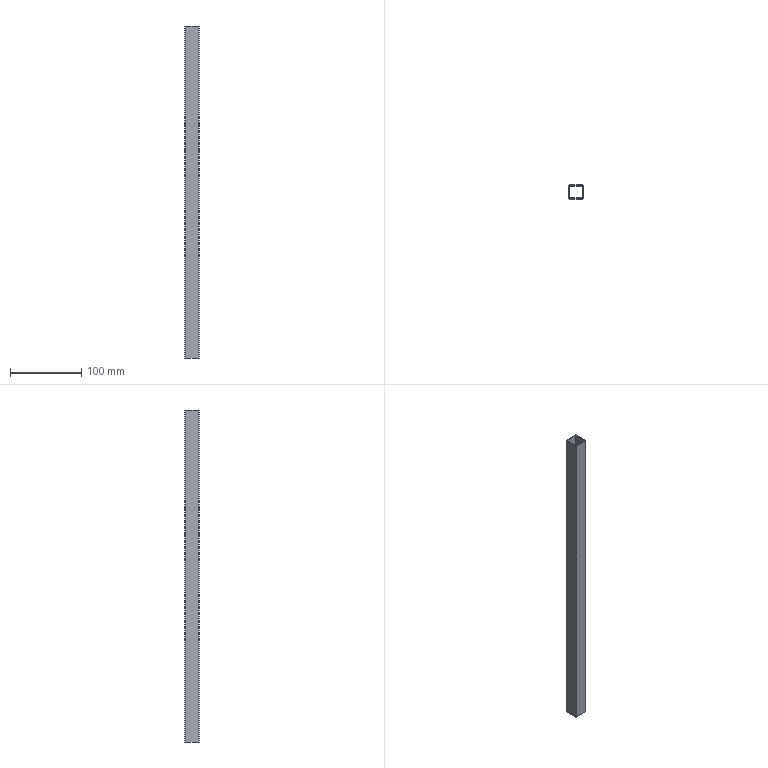Component | SolidWorks | Stiffener-1 | 1 solid | 14 faces | box 20 x 20 x 467.6 mm | volume 41795 mm3 | plane 10 | cylinder 4 | commonest cylinder face diameters 2 x4
build123d program:
from build123d import *

# Parameters (mm, degrees)
SKETCH1_W           = 17.6
SKETCH1_H           = 17.6
BOSS_EXTRUDE1_DEPTH = 467.6


with BuildPart() as part:
    # Sketch1 → Boss-Extrude1 (new body)
    with BuildSketch(Plane.XY):
        with BuildLine():
            Line((-75.47, 58.704), (-57.47, 58.704))
            ThreePointArc((-57.47, 58.704), (-56.763, 58.411), (-56.47, 57.704))
            Line((-56.47, 57.704), (-56.47, 39.704))
            ThreePointArc((-56.47, 39.704), (-56.763, 38.997), (-57.47, 38.704))
            Line((-57.47, 38.704), (-75.47, 38.704))
            ThreePointArc((-75.47, 38.704), (-76.177, 38.997), (-76.47, 39.704))
            Line((-76.47, 39.704), (-76.47, 57.704))
            ThreePointArc((-76.47, 57.704), (-76.177, 58.411), (-75.47, 58.704))
        make_face()
        with Locations((-66.47, 48.704)):
            Rectangle(SKETCH1_W, SKETCH1_H, mode=Mode.SUBTRACT)
    extrude(amount=BOSS_EXTRUDE1_DEPTH)


solid = part.part

# Placed as in the assembly
solid = solid.moved(Location((274.97, 197.296, -115.8), (0, 0, 0)))
STEP:
#1=CARTESIAN_POINT('',(8.563,9.291,13.85));
#2=VERTEX_POINT('',#1);
#3=CARTESIAN_POINT('',(8.602,9.331,13.85));
#4=VERTEX_POINT('',#3);
#5=CARTESIAN_POINT('',(8.563,9.331,13.85));
#6=DIRECTION('',(-0.,0.,1.));
#7=DIRECTION('',(-1.,0.,0.));
#8=AXIS2_PLACEMENT_3D('',#5,#6,#7);
#9=CIRCLE('',#8,0.03937);
#10=EDGE_CURVE('',#2,#4,#9,.T.);
#11=ORIENTED_EDGE('',*,*,#10,.T.);
#12=CARTESIAN_POINT('',(8.602,10.039,13.85));
#13=VERTEX_POINT('',#12);
#14=CARTESIAN_POINT('',(8.602,9.331,13.85));
#15=DIRECTION('',(-0.,1.,-0.));
#16=VECTOR('',#15,39.37);
#17=LINE('',#14,#16);
#18=EDGE_CURVE('',#4,#13,#17,.T.);
#19=ORIENTED_EDGE('',*,*,#18,.T.);
#20=CARTESIAN_POINT('',(8.563,10.079,13.85));
#21=VERTEX_POINT('',#20);
#22=CARTESIAN_POINT('',(8.563,10.039,13.85));
#23=DIRECTION('',(-0.,0.,1.));
#24=DIRECTION('',(1.,0.,0.));
#25=AXIS2_PLACEMENT_3D('',#22,#23,#24);
#26=CIRCLE('',#25,0.03937);
#27=EDGE_CURVE('',#13,#21,#26,.T.);
#28=ORIENTED_EDGE('',*,*,#27,.T.);
#29=CARTESIAN_POINT('',(7.854,10.079,13.85));
#30=VERTEX_POINT('',#29);
#31=CARTESIAN_POINT('',(8.563,10.079,13.85));
#32=DIRECTION('',(-1.,0.,-0.));
#33=VECTOR('',#32,39.37);
#34=LINE('',#31,#33);
#35=EDGE_CURVE('',#21,#30,#34,.T.);
#36=ORIENTED_EDGE('',*,*,#35,.T.);
#37=CARTESIAN_POINT('',(7.815,10.039,13.85));
#38=VERTEX_POINT('',#37);
#39=CARTESIAN_POINT('',(7.854,10.039,13.85));
#40=DIRECTION('',(-0.,0.,1.));
#41=DIRECTION('',(-1.,0.,0.));
#42=AXIS2_PLACEMENT_3D('',#39,#40,#41);
#43=CIRCLE('',#42,0.03937);
#44=EDGE_CURVE('',#30,#38,#43,.T.);
#45=ORIENTED_EDGE('',*,*,#44,.T.);
#46=CARTESIAN_POINT('',(7.815,9.331,13.85));
#47=VERTEX_POINT('',#46);
#48=CARTESIAN_POINT('',(7.815,9.331,13.85));
#49=DIRECTION('',(-0.,-1.,0.));
#50=VECTOR('',#49,39.37);
#51=LINE('',#48,#50);
#52=EDGE_CURVE('',#38,#47,#51,.T.);
#53=ORIENTED_EDGE('',*,*,#52,.T.);
#54=CARTESIAN_POINT('',(7.854,9.291,13.85));
#55=VERTEX_POINT('',#54);
#56=CARTESIAN_POINT('',(7.854,9.331,13.85));
#57=DIRECTION('',(-0.,0.,1.));
#58=DIRECTION('',(-1.,0.,0.));
#59=AXIS2_PLACEMENT_3D('',#56,#57,#58);
#60=CIRCLE('',#59,0.03937);
#61=EDGE_CURVE('',#47,#55,#60,.T.);
#62=ORIENTED_EDGE('',*,*,#61,.T.);
#63=CARTESIAN_POINT('',(8.563,9.291,13.85));
#64=DIRECTION('',(1.,-0.,0.));
#65=VECTOR('',#64,39.37);
#66=LINE('',#63,#65);
#67=EDGE_CURVE('',#55,#2,#66,.T.);
#68=ORIENTED_EDGE('',*,*,#67,.T.);
#69=EDGE_LOOP('',(#11,#19,#28,#36,#45,#53,#62,#68));
#70=FACE_OUTER_BOUND('',#69,.T.);
#71=CARTESIAN_POINT('',(8.555,9.339,13.85));
#72=VERTEX_POINT('',#71);
#73=CARTESIAN_POINT('',(8.555,10.031,13.85));
#74=VERTEX_POINT('',#73);
#75=CARTESIAN_POINT('',(8.555,9.339,13.85));
#76=DIRECTION('',(0.,1.,-0.));
#77=VECTOR('',#76,39.37);
#78=LINE('',#75,#77);
#79=EDGE_CURVE('',#72,#74,#78,.T.);
#80=ORIENTED_EDGE('',*,*,#79,.F.);
#81=CARTESIAN_POINT('',(7.862,9.339,13.85));
#82=VERTEX_POINT('',#81);
#83=CARTESIAN_POINT('',(8.555,9.339,13.85));
#84=DIRECTION('',(1.,-0.,0.));
#85=VECTOR('',#84,39.37);
#86=LINE('',#83,#85);
#87=EDGE_CURVE('',#82,#72,#86,.T.);
#88=ORIENTED_EDGE('',*,*,#87,.F.);
#89=CARTESIAN_POINT('',(7.862,10.031,13.85));
#90=VERTEX_POINT('',#89);
#91=CARTESIAN_POINT('',(7.862,9.339,13.85));
#92=DIRECTION('',(-0.,-1.,0.));
#93=VECTOR('',#92,39.37);
#94=LINE('',#91,#93);
#95=EDGE_CURVE('',#90,#82,#94,.T.);
#96=ORIENTED_EDGE('',*,*,#95,.F.);
#97=CARTESIAN_POINT('',(8.555,10.031,13.85));
#98=DIRECTION('',(-1.,0.,-0.));
#99=VECTOR('',#98,39.37);
#100=LINE('',#97,#99);
#101=EDGE_CURVE('',#74,#90,#100,.T.);
#102=ORIENTED_EDGE('',*,*,#101,.F.);
#103=EDGE_LOOP('',(#80,#88,#96,#102));
#104=FACE_BOUND('',#103,.T.);
#105=CARTESIAN_POINT('',(8.563,9.331,13.85));
#106=DIRECTION('',(-0.,0.,1.));
#107=DIRECTION('',(-1.,0.,-0.));
#108=AXIS2_PLACEMENT_3D('',#105,#106,#107);
#109=PLANE('',#108);
#110=ADVANCED_FACE('',(#70,#104),#109,.T.);
#111=CARTESIAN_POINT('',(8.563,9.291,-4.559));
#112=VERTEX_POINT('',#111);
#113=CARTESIAN_POINT('',(8.602,9.331,-4.559));
#114=VERTEX_POINT('',#113);
#115=CARTESIAN_POINT('',(8.563,9.331,-4.559));
#116=DIRECTION('',(-0.,0.,1.));
#117=DIRECTION('',(-1.,0.,0.));
#118=AXIS2_PLACEMENT_3D('',#115,#116,#117);
#119=CIRCLE('',#118,0.03937);
#120=EDGE_CURVE('',#112,#114,#119,.T.);
#121=ORIENTED_EDGE('',*,*,#120,.F.);
#122=CARTESIAN_POINT('',(7.854,9.291,-4.559));
#123=VERTEX_POINT('',#122);
#124=CARTESIAN_POINT('',(8.563,9.291,-4.559));
#125=DIRECTION('',(1.,-0.,0.));
#126=VECTOR('',#125,39.37);
#127=LINE('',#124,#126);
#128=EDGE_CURVE('',#123,#112,#127,.T.);
#129=ORIENTED_EDGE('',*,*,#128,.F.);
#130=CARTESIAN_POINT('',(7.815,9.331,-4.559));
#131=VERTEX_POINT('',#130);
#132=CARTESIAN_POINT('',(7.854,9.331,-4.559));
#133=DIRECTION('',(-0.,0.,1.));
#134=DIRECTION('',(-1.,0.,0.));
#135=AXIS2_PLACEMENT_3D('',#132,#133,#134);
#136=CIRCLE('',#135,0.03937);
#137=EDGE_CURVE('',#131,#123,#136,.T.);
#138=ORIENTED_EDGE('',*,*,#137,.F.);
#139=CARTESIAN_POINT('',(7.815,10.039,-4.559));
#140=VERTEX_POINT('',#139);
#141=CARTESIAN_POINT('',(7.815,9.331,-4.559));
#142=DIRECTION('',(-0.,-1.,0.));
#143=VECTOR('',#142,39.37);
#144=LINE('',#141,#143);
#145=EDGE_CURVE('',#140,#131,#144,.T.);
#146=ORIENTED_EDGE('',*,*,#145,.F.);
#147=CARTESIAN_POINT('',(7.854,10.079,-4.559));
#148=VERTEX_POINT('',#147);
#149=CARTESIAN_POINT('',(7.854,10.039,-4.559));
#150=DIRECTION('',(-0.,0.,1.));
#151=DIRECTION('',(-1.,0.,0.));
#152=AXIS2_PLACEMENT_3D('',#149,#150,#151);
#153=CIRCLE('',#152,0.03937);
#154=EDGE_CURVE('',#148,#140,#153,.T.);
#155=ORIENTED_EDGE('',*,*,#154,.F.);
#156=CARTESIAN_POINT('',(8.563,10.079,-4.559));
#157=VERTEX_POINT('',#156);
#158=CARTESIAN_POINT('',(8.563,10.079,-4.559));
#159=DIRECTION('',(-1.,0.,-0.));
#160=VECTOR('',#159,39.37);
#161=LINE('',#158,#160);
#162=EDGE_CURVE('',#157,#148,#161,.T.);
#163=ORIENTED_EDGE('',*,*,#162,.F.);
#164=CARTESIAN_POINT('',(8.602,10.039,-4.559));
#165=VERTEX_POINT('',#164);
#166=CARTESIAN_POINT('',(8.563,10.039,-4.559));
#167=DIRECTION('',(-0.,0.,1.));
#168=DIRECTION('',(1.,0.,0.));
#169=AXIS2_PLACEMENT_3D('',#166,#167,#168);
#170=CIRCLE('',#169,0.03937);
#171=EDGE_CURVE('',#165,#157,#170,.T.);
#172=ORIENTED_EDGE('',*,*,#171,.F.);
#173=CARTESIAN_POINT('',(8.602,9.331,-4.559));
#174=DIRECTION('',(-0.,1.,-0.));
#175=VECTOR('',#174,39.37);
#176=LINE('',#173,#175);
#177=EDGE_CURVE('',#114,#165,#176,.T.);
#178=ORIENTED_EDGE('',*,*,#177,.F.);
#179=EDGE_LOOP('',(#121,#129,#138,#146,#155,#163,#172,#178));
#180=FACE_OUTER_BOUND('',#179,.T.);
#181=CARTESIAN_POINT('',(7.862,9.339,-4.559));
#182=VERTEX_POINT('',#181);
#183=CARTESIAN_POINT('',(8.555,9.339,-4.559));
#184=VERTEX_POINT('',#183);
#185=CARTESIAN_POINT('',(8.555,9.339,-4.559));
#186=DIRECTION('',(1.,-0.,0.));
#187=VECTOR('',#186,39.37);
#188=LINE('',#185,#187);
#189=EDGE_CURVE('',#182,#184,#188,.T.);
#190=ORIENTED_EDGE('',*,*,#189,.T.);
#191=CARTESIAN_POINT('',(8.555,10.031,-4.559));
#192=VERTEX_POINT('',#191);
#193=CARTESIAN_POINT('',(8.555,9.339,-4.559));
#194=DIRECTION('',(0.,1.,-0.));
#195=VECTOR('',#194,39.37);
#196=LINE('',#193,#195);
#197=EDGE_CURVE('',#184,#192,#196,.T.);
#198=ORIENTED_EDGE('',*,*,#197,.T.);
#199=CARTESIAN_POINT('',(7.862,10.031,-4.559));
#200=VERTEX_POINT('',#199);
#201=CARTESIAN_POINT('',(8.555,10.031,-4.559));
#202=DIRECTION('',(-1.,0.,-0.));
#203=VECTOR('',#202,39.37);
#204=LINE('',#201,#203);
#205=EDGE_CURVE('',#192,#200,#204,.T.);
#206=ORIENTED_EDGE('',*,*,#205,.T.);
#207=CARTESIAN_POINT('',(7.862,9.339,-4.559));
#208=DIRECTION('',(-0.,-1.,0.));
#209=VECTOR('',#208,39.37);
#210=LINE('',#207,#209);
#211=EDGE_CURVE('',#200,#182,#210,.T.);
#212=ORIENTED_EDGE('',*,*,#211,.T.);
#213=EDGE_LOOP('',(#190,#198,#206,#212));
#214=FACE_BOUND('',#213,.T.);
#215=CARTESIAN_POINT('',(8.563,9.331,-4.559));
#216=DIRECTION('',(-0.,0.,1.));
#217=DIRECTION('',(-1.,0.,-0.));
#218=AXIS2_PLACEMENT_3D('',#215,#216,#217);
#219=PLANE('',#218);
#220=ADVANCED_FACE('',(#180,#214),#219,.F.);
#221=ORIENTED_EDGE('',*,*,#120,.T.);
#222=CARTESIAN_POINT('',(8.602,9.331,13.85));
#223=DIRECTION('',(0.,-0.,-1.));
#224=VECTOR('',#223,39.37);
#225=LINE('',#222,#224);
#226=EDGE_CURVE('',#4,#114,#225,.T.);
#227=ORIENTED_EDGE('',*,*,#226,.F.);
#228=ORIENTED_EDGE('',*,*,#10,.F.);
#229=CARTESIAN_POINT('',(8.563,9.291,13.85));
#230=DIRECTION('',(0.,-0.,-1.));
#231=VECTOR('',#230,39.37);
#232=LINE('',#229,#231);
#233=EDGE_CURVE('',#2,#112,#232,.T.);
#234=ORIENTED_EDGE('',*,*,#233,.T.);
#235=EDGE_LOOP('',(#221,#227,#228,#234));
#236=FACE_OUTER_BOUND('',#235,.T.);
#237=CARTESIAN_POINT('',(8.563,9.331,13.85));
#238=DIRECTION('',(0.,-0.,-1.));
#239=DIRECTION('',(1.,0.,0.));
#240=AXIS2_PLACEMENT_3D('',#237,#238,#239);
#241=CYLINDRICAL_SURFACE('',#240,0.03937);
#242=ADVANCED_FACE('',(#236),#241,.T.);
#243=ORIENTED_EDGE('',*,*,#177,.T.);
#244=CARTESIAN_POINT('',(8.602,10.039,13.85));
#245=DIRECTION('',(0.,-0.,-1.));
#246=VECTOR('',#245,39.37);
#247=LINE('',#244,#246);
#248=EDGE_CURVE('',#13,#165,#247,.T.);
#249=ORIENTED_EDGE('',*,*,#248,.F.);
#250=ORIENTED_EDGE('',*,*,#18,.F.);
#251=ORIENTED_EDGE('',*,*,#226,.T.);
#252=EDGE_LOOP('',(#243,#249,#250,#251));
#253=FACE_OUTER_BOUND('',#252,.T.);
#254=CARTESIAN_POINT('',(8.602,9.331,13.85));
#255=DIRECTION('',(-1.,-0.,-0.));
#256=DIRECTION('',(0.,-1.,0.));
#257=AXIS2_PLACEMENT_3D('',#254,#255,#256);
#258=PLANE('',#257);
#259=ADVANCED_FACE('',(#253),#258,.F.);
#260=ORIENTED_EDGE('',*,*,#171,.T.);
#261=CARTESIAN_POINT('',(8.563,10.079,13.85));
#262=DIRECTION('',(0.,-0.,-1.));
#263=VECTOR('',#262,39.37);
#264=LINE('',#261,#263);
#265=EDGE_CURVE('',#21,#157,#264,.T.);
#266=ORIENTED_EDGE('',*,*,#265,.F.);
#267=ORIENTED_EDGE('',*,*,#27,.F.);
#268=ORIENTED_EDGE('',*,*,#248,.T.);
#269=EDGE_LOOP('',(#260,#266,#267,#268));
#270=FACE_OUTER_BOUND('',#269,.T.);
#271=CARTESIAN_POINT('',(8.563,10.039,13.85));
#272=DIRECTION('',(0.,-0.,-1.));
#273=DIRECTION('',(1.,0.,0.));
#274=AXIS2_PLACEMENT_3D('',#271,#272,#273);
#275=CYLINDRICAL_SURFACE('',#274,0.03937);
#276=ADVANCED_FACE('',(#270),#275,.T.);
#277=ORIENTED_EDGE('',*,*,#162,.T.);
#278=CARTESIAN_POINT('',(7.854,10.079,13.85));
#279=DIRECTION('',(0.,-0.,-1.));
#280=VECTOR('',#279,39.37);
#281=LINE('',#278,#280);
#282=EDGE_CURVE('',#30,#148,#281,.T.);
#283=ORIENTED_EDGE('',*,*,#282,.F.);
#284=ORIENTED_EDGE('',*,*,#35,.F.);
#285=ORIENTED_EDGE('',*,*,#265,.T.);
#286=EDGE_LOOP('',(#277,#283,#284,#285));
#287=FACE_OUTER_BOUND('',#286,.T.);
#288=CARTESIAN_POINT('',(8.563,10.079,13.85));
#289=DIRECTION('',(-0.,-1.,0.));
#290=DIRECTION('',(-0.,0.,1.));
#291=AXIS2_PLACEMENT_3D('',#288,#289,#290);
#292=PLANE('',#291);
#293=ADVANCED_FACE('',(#287),#292,.F.);
#294=ORIENTED_EDGE('',*,*,#154,.T.);
#295=CARTESIAN_POINT('',(7.815,10.039,13.85));
#296=DIRECTION('',(0.,-0.,-1.));
#297=VECTOR('',#296,39.37);
#298=LINE('',#295,#297);
#299=EDGE_CURVE('',#38,#140,#298,.T.);
#300=ORIENTED_EDGE('',*,*,#299,.F.);
#301=ORIENTED_EDGE('',*,*,#44,.F.);
#302=ORIENTED_EDGE('',*,*,#282,.T.);
#303=EDGE_LOOP('',(#294,#300,#301,#302));
#304=FACE_OUTER_BOUND('',#303,.T.);
#305=CARTESIAN_POINT('',(7.854,10.039,13.85));
#306=DIRECTION('',(0.,-0.,-1.));
#307=DIRECTION('',(1.,0.,0.));
#308=AXIS2_PLACEMENT_3D('',#305,#306,#307);
#309=CYLINDRICAL_SURFACE('',#308,0.03937);
#310=ADVANCED_FACE('',(#304),#309,.T.);
#311=ORIENTED_EDGE('',*,*,#145,.T.);
#312=CARTESIAN_POINT('',(7.815,9.331,13.85));
#313=DIRECTION('',(0.,-0.,-1.));
#314=VECTOR('',#313,39.37);
#315=LINE('',#312,#314);
#316=EDGE_CURVE('',#47,#131,#315,.T.);
#317=ORIENTED_EDGE('',*,*,#316,.F.);
#318=ORIENTED_EDGE('',*,*,#52,.F.);
#319=ORIENTED_EDGE('',*,*,#299,.T.);
#320=EDGE_LOOP('',(#311,#317,#318,#319));
#321=FACE_OUTER_BOUND('',#320,.T.);
#322=CARTESIAN_POINT('',(7.815,9.331,13.85));
#323=DIRECTION('',(1.,-0.,0.));
#324=DIRECTION('',(0.,1.,-0.));
#325=AXIS2_PLACEMENT_3D('',#322,#323,#324);
#326=PLANE('',#325);
#327=ADVANCED_FACE('',(#321),#326,.F.);
#328=ORIENTED_EDGE('',*,*,#137,.T.);
#329=CARTESIAN_POINT('',(7.854,9.291,13.85));
#330=DIRECTION('',(0.,-0.,-1.));
#331=VECTOR('',#330,39.37);
#332=LINE('',#329,#331);
#333=EDGE_CURVE('',#55,#123,#332,.T.);
#334=ORIENTED_EDGE('',*,*,#333,.F.);
#335=ORIENTED_EDGE('',*,*,#61,.F.);
#336=ORIENTED_EDGE('',*,*,#316,.T.);
#337=EDGE_LOOP('',(#328,#334,#335,#336));
#338=FACE_OUTER_BOUND('',#337,.T.);
#339=CARTESIAN_POINT('',(7.854,9.331,13.85));
#340=DIRECTION('',(0.,-0.,-1.));
#341=DIRECTION('',(1.,0.,0.));
#342=AXIS2_PLACEMENT_3D('',#339,#340,#341);
#343=CYLINDRICAL_SURFACE('',#342,0.03937);
#344=ADVANCED_FACE('',(#338),#343,.T.);
#345=ORIENTED_EDGE('',*,*,#128,.T.);
#346=ORIENTED_EDGE('',*,*,#233,.F.);
#347=ORIENTED_EDGE('',*,*,#67,.F.);
#348=ORIENTED_EDGE('',*,*,#333,.T.);
#349=EDGE_LOOP('',(#345,#346,#347,#348));
#350=FACE_OUTER_BOUND('',#349,.T.);
#351=CARTESIAN_POINT('',(8.563,9.291,13.85));
#352=DIRECTION('',(0.,1.,-0.));
#353=DIRECTION('',(0.,-0.,-1.));
#354=AXIS2_PLACEMENT_3D('',#351,#352,#353);
#355=PLANE('',#354);
#356=ADVANCED_FACE('',(#350),#355,.F.);
#357=ORIENTED_EDGE('',*,*,#189,.F.);
#358=CARTESIAN_POINT('',(7.862,9.339,13.85));
#359=DIRECTION('',(0.,-0.,-1.));
#360=VECTOR('',#359,39.37);
#361=LINE('',#358,#360);
#362=EDGE_CURVE('',#82,#182,#361,.T.);
#363=ORIENTED_EDGE('',*,*,#362,.F.);
#364=ORIENTED_EDGE('',*,*,#87,.T.);
#365=CARTESIAN_POINT('',(8.555,9.339,13.85));
#366=DIRECTION('',(0.,-0.,-1.));
#367=VECTOR('',#366,39.37);
#368=LINE('',#365,#367);
#369=EDGE_CURVE('',#72,#184,#368,.T.);
#370=ORIENTED_EDGE('',*,*,#369,.T.);
#371=EDGE_LOOP('',(#357,#363,#364,#370));
#372=FACE_OUTER_BOUND('',#371,.T.);
#373=CARTESIAN_POINT('',(8.555,9.339,13.85));
#374=DIRECTION('',(0.,1.,-0.));
#375=DIRECTION('',(0.,-0.,-1.));
#376=AXIS2_PLACEMENT_3D('',#373,#374,#375);
#377=PLANE('',#376);
#378=ADVANCED_FACE('',(#372),#377,.T.);
#379=ORIENTED_EDGE('',*,*,#197,.F.);
#380=ORIENTED_EDGE('',*,*,#369,.F.);
#381=ORIENTED_EDGE('',*,*,#79,.T.);
#382=CARTESIAN_POINT('',(8.555,10.031,13.85));
#383=DIRECTION('',(0.,-0.,-1.));
#384=VECTOR('',#383,39.37);
#385=LINE('',#382,#384);
#386=EDGE_CURVE('',#74,#192,#385,.T.);
#387=ORIENTED_EDGE('',*,*,#386,.T.);
#388=EDGE_LOOP('',(#379,#380,#381,#387));
#389=FACE_OUTER_BOUND('',#388,.T.);
#390=CARTESIAN_POINT('',(8.555,9.339,13.85));
#391=DIRECTION('',(-1.,0.,-0.));
#392=DIRECTION('',(0.,-0.,-1.));
#393=AXIS2_PLACEMENT_3D('',#390,#391,#392);
#394=PLANE('',#393);
#395=ADVANCED_FACE('',(#389),#394,.T.);
#396=ORIENTED_EDGE('',*,*,#205,.F.);
#397=ORIENTED_EDGE('',*,*,#386,.F.);
#398=ORIENTED_EDGE('',*,*,#101,.T.);
#399=CARTESIAN_POINT('',(7.862,10.031,13.85));
#400=DIRECTION('',(0.,-0.,-1.));
#401=VECTOR('',#400,39.37);
#402=LINE('',#399,#401);
#403=EDGE_CURVE('',#90,#200,#402,.T.);
#404=ORIENTED_EDGE('',*,*,#403,.T.);
#405=EDGE_LOOP('',(#396,#397,#398,#404));
#406=FACE_OUTER_BOUND('',#405,.T.);
#407=CARTESIAN_POINT('',(8.555,10.031,13.85));
#408=DIRECTION('',(-0.,-1.,0.));
#409=DIRECTION('',(-0.,0.,1.));
#410=AXIS2_PLACEMENT_3D('',#407,#408,#409);
#411=PLANE('',#410);
#412=ADVANCED_FACE('',(#406),#411,.T.);
#413=ORIENTED_EDGE('',*,*,#211,.F.);
#414=ORIENTED_EDGE('',*,*,#403,.F.);
#415=ORIENTED_EDGE('',*,*,#95,.T.);
#416=ORIENTED_EDGE('',*,*,#362,.T.);
#417=EDGE_LOOP('',(#413,#414,#415,#416));
#418=FACE_OUTER_BOUND('',#417,.T.);
#419=CARTESIAN_POINT('',(7.862,9.339,13.85));
#420=DIRECTION('',(1.,-0.,0.));
#421=DIRECTION('',(-0.,0.,1.));
#422=AXIS2_PLACEMENT_3D('',#419,#420,#421);
#423=PLANE('',#422);
#424=ADVANCED_FACE('',(#418),#423,.T.);
#425=CLOSED_SHELL('',(#110,#220,#242,#259,#276,#293,#310,#327,#344,#356,#378,#395,#412,#424));
#426=MANIFOLD_SOLID_BREP('',#425);
#427=CARTESIAN_POINT('',(0.,0.,0.));
#428=DIRECTION('',(0.,0.,1.));
#429=DIRECTION('',(1.,0.,0.));
#430=AXIS2_PLACEMENT_3D('',#427,#428,#429);
#431=(LENGTH_UNIT()NAMED_UNIT(*)SI_UNIT($,.METRE.));
#432=LENGTH_MEASURE_WITH_UNIT(LENGTH_MEASURE(0.0254),#431);
#433=DIMENSIONAL_EXPONENTS(1.,0.,0.,0.,0.,0.,0.);
#434=(CONVERSION_BASED_UNIT('',#432)LENGTH_UNIT()NAMED_UNIT(#433));
#435=UNCERTAINTY_MEASURE_WITH_UNIT(LENGTH_MEASURE(0.00001),#434,'','');
#436=(NAMED_UNIT(*)PLANE_ANGLE_UNIT()SI_UNIT($,.RADIAN.));
#437=(NAMED_UNIT(*)SI_UNIT($,.STERADIAN.)SOLID_ANGLE_UNIT());
#438=(GEOMETRIC_REPRESENTATION_CONTEXT(3)GLOBAL_UNCERTAINTY_ASSIGNED_CONTEXT((#435))GLOBAL_UNIT_ASSIGNED_CONTEXT((#434,#436,#437))REPRESENTATION_CONTEXT('',''));
#439=ADVANCED_BREP_SHAPE_REPRESENTATION('',(#426,#430),#438);
#440=COLOUR_RGB('',0.7922,0.8196,0.9333);
#441=FILL_AREA_STYLE_COLOUR('',#440);
#442=FILL_AREA_STYLE('',(#441));
#443=SURFACE_STYLE_FILL_AREA(#442);
#444=SURFACE_SIDE_STYLE('',(#443));
#445=SURFACE_STYLE_USAGE(.BOTH.,#444);
#446=PRESENTATION_STYLE_ASSIGNMENT((#445));
#447=STYLED_ITEM('',(#446),#426);
#448=(LENGTH_UNIT()NAMED_UNIT(*)SI_UNIT($,.METRE.));
#449=LENGTH_MEASURE_WITH_UNIT(LENGTH_MEASURE(0.0254),#448);
#450=DIMENSIONAL_EXPONENTS(1.,0.,0.,0.,0.,0.,0.);
#451=(CONVERSION_BASED_UNIT('',#449)LENGTH_UNIT()NAMED_UNIT(#450));
#452=UNCERTAINTY_MEASURE_WITH_UNIT(LENGTH_MEASURE(0.00001),#451,'','');
#453=(NAMED_UNIT(*)PLANE_ANGLE_UNIT()SI_UNIT($,.RADIAN.));
#454=(NAMED_UNIT(*)SI_UNIT($,.STERADIAN.)SOLID_ANGLE_UNIT());
#455=(GEOMETRIC_REPRESENTATION_CONTEXT(3)GLOBAL_UNCERTAINTY_ASSIGNED_CONTEXT((#452))GLOBAL_UNIT_ASSIGNED_CONTEXT((#451,#453,#454))REPRESENTATION_CONTEXT('',''));
#456=MECHANICAL_DESIGN_GEOMETRIC_PRESENTATION_REPRESENTATION('',(#447),#455);
#457=PRESENTATION_LAYER_ASSIGNMENT('','',(#447));